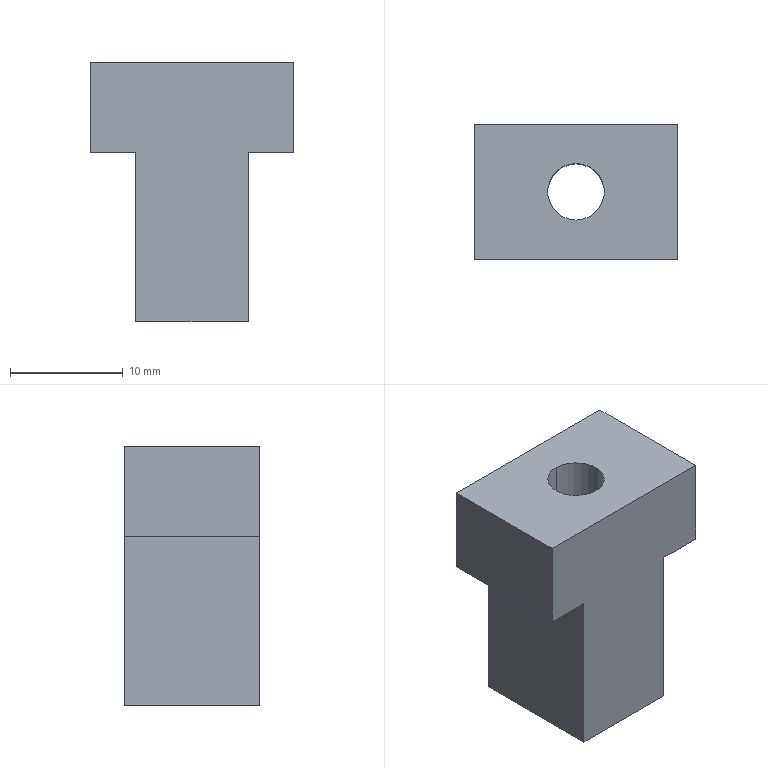Component | SolidWorks | SecondGenerationFour-sidedLabelingFeedingCylinderConnector-1 | 1 solid | 12 faces | box 18 x 12 x 23 mm | volume 3076 mm3 | plane 10 | cylinder 2 | commonest cylinder face diameters 5 x2
build123d program:
from build123d import *

# Parameters (mm, degrees)
SKETCH1_W             = 18
SKETCH1_H             = 8
BOSS_EXTRUDE1_DEPTH   = 6
SKETCH2_W             = 10
SKETCH2_H             = 12
BOSS_EXTRUDE2_DEPTH   = 15
M6_TAPPED_HOLE1_D     = 5
M6_TAPPED_HOLE1_DEPTH = 25
M6_TAPPED_HOLE1_TIP   = 1.502


with BuildPart() as part:
    # Sketch1 → Boss-Extrude1 (new, symmetric)
    with BuildSketch(Plane.XY):
        Rectangle(SKETCH1_W, SKETCH1_H)
    extrude(amount=BOSS_EXTRUDE1_DEPTH, both=True)

    # Sketch2 → Boss-Extrude2 (add)
    with BuildSketch(Plane(origin=(0, 4, 0), x_dir=(1, 0, 0), z_dir=(0, 1, 0))):
        Rectangle(SKETCH2_W, SKETCH2_H)
    extrude(amount=BOSS_EXTRUDE2_DEPTH)

    # M6 Tapped Hole1
    with Locations(Plane(origin=(0, 19, 0), x_dir=(-1, 0, 0), z_dir=(0, 1, 0))):
        with Locations((0, 0)):
            Hole(M6_TAPPED_HOLE1_D / 2, depth=M6_TAPPED_HOLE1_DEPTH)
            with Locations((0, 0, -(M6_TAPPED_HOLE1_DEPTH + M6_TAPPED_HOLE1_TIP / 2))):  # 118° drill point
                Cone(0, M6_TAPPED_HOLE1_D / 2, M6_TAPPED_HOLE1_TIP, mode=Mode.SUBTRACT)


solid = part.part

# Placed as in the assembly
solid = solid.moved(Location((59.973, -16.137, -142.5), (-90, 0, 0)))
STEP:
#1=CARTESIAN_POINT('',(2.361,-0.7337,-5.453));
#2=VERTEX_POINT('',#1);
#3=CARTESIAN_POINT('',(2.361,-0.5369,-5.453));
#4=VERTEX_POINT('',#3);
#5=CARTESIAN_POINT('',(2.361,-0.6353,-5.453));
#6=DIRECTION('',(-0.,-0.,-1.));
#7=DIRECTION('',(0.,1.,0.));
#8=AXIS2_PLACEMENT_3D('',#5,#6,#7);
#9=CIRCLE('',#8,0.09843);
#10=EDGE_CURVE('',#2,#4,#9,.T.);
#11=ORIENTED_EDGE('',*,*,#10,.F.);
#12=CARTESIAN_POINT('',(2.361,-0.7337,-6.358));
#13=VERTEX_POINT('',#12);
#14=CARTESIAN_POINT('',(2.361,-0.7337,-6.358));
#15=DIRECTION('',(-0.,-0.,-1.));
#16=VECTOR('',#15,39.37);
#17=LINE('',#14,#16);
#18=EDGE_CURVE('',#2,#13,#17,.T.);
#19=ORIENTED_EDGE('',*,*,#18,.T.);
#20=CARTESIAN_POINT('',(2.361,-0.5369,-6.358));
#21=VERTEX_POINT('',#20);
#22=CARTESIAN_POINT('',(2.361,-0.6353,-6.358));
#23=DIRECTION('',(-0.,-0.,-1.));
#24=DIRECTION('',(0.,1.,0.));
#25=AXIS2_PLACEMENT_3D('',#22,#23,#24);
#26=CIRCLE('',#25,0.09843);
#27=EDGE_CURVE('',#13,#21,#26,.T.);
#28=ORIENTED_EDGE('',*,*,#27,.T.);
#29=CARTESIAN_POINT('',(2.361,-0.5369,-6.358));
#30=DIRECTION('',(-0.,-0.,-1.));
#31=VECTOR('',#30,39.37);
#32=LINE('',#29,#31);
#33=EDGE_CURVE('',#4,#21,#32,.T.);
#34=ORIENTED_EDGE('',*,*,#33,.F.);
#35=EDGE_LOOP('',(#11,#19,#28,#34));
#36=FACE_OUTER_BOUND('',#35,.T.);
#37=CARTESIAN_POINT('',(2.361,-0.6353,-6.358));
#38=DIRECTION('',(-0.,-0.,-1.));
#39=DIRECTION('',(0.,1.,0.));
#40=AXIS2_PLACEMENT_3D('',#37,#38,#39);
#41=CYLINDRICAL_SURFACE('',#40,0.09843);
#42=ADVANCED_FACE('',(#36),#41,.F.);
#43=CARTESIAN_POINT('',(2.558,-0.3991,-5.768));
#44=VERTEX_POINT('',#43);
#45=CARTESIAN_POINT('',(2.558,-0.8715,-5.768));
#46=VERTEX_POINT('',#45);
#47=CARTESIAN_POINT('',(2.558,-0.3991,-5.768));
#48=DIRECTION('',(-0.,-1.,0.));
#49=VECTOR('',#48,39.37);
#50=LINE('',#47,#49);
#51=EDGE_CURVE('',#44,#46,#50,.T.);
#52=ORIENTED_EDGE('',*,*,#51,.F.);
#53=CARTESIAN_POINT('',(2.715,-0.3991,-5.768));
#54=VERTEX_POINT('',#53);
#55=CARTESIAN_POINT('',(2.007,-0.3991,-5.768));
#56=DIRECTION('',(-1.,0.,0.));
#57=VECTOR('',#56,39.37);
#58=LINE('',#55,#57);
#59=EDGE_CURVE('',#54,#44,#58,.T.);
#60=ORIENTED_EDGE('',*,*,#59,.F.);
#61=CARTESIAN_POINT('',(2.715,-0.8715,-5.768));
#62=VERTEX_POINT('',#61);
#63=CARTESIAN_POINT('',(2.715,-0.3991,-5.768));
#64=DIRECTION('',(-0.,-1.,0.));
#65=VECTOR('',#64,39.37);
#66=LINE('',#63,#65);
#67=EDGE_CURVE('',#54,#62,#66,.T.);
#68=ORIENTED_EDGE('',*,*,#67,.T.);
#69=CARTESIAN_POINT('',(2.007,-0.8715,-5.768));
#70=DIRECTION('',(-1.,0.,0.));
#71=VECTOR('',#70,39.37);
#72=LINE('',#69,#71);
#73=EDGE_CURVE('',#62,#46,#72,.T.);
#74=ORIENTED_EDGE('',*,*,#73,.T.);
#75=EDGE_LOOP('',(#52,#60,#68,#74));
#76=FACE_OUTER_BOUND('',#75,.T.);
#77=CARTESIAN_POINT('',(2.007,-0.3991,-5.768));
#78=DIRECTION('',(0.,0.,1.));
#79=DIRECTION('',(-0.,-1.,0.));
#80=AXIS2_PLACEMENT_3D('',#77,#78,#79);
#81=PLANE('',#80);
#82=ADVANCED_FACE('',(#76),#81,.F.);
#83=CARTESIAN_POINT('',(2.164,-0.8715,-5.768));
#84=VERTEX_POINT('',#83);
#85=CARTESIAN_POINT('',(2.164,-0.3991,-5.768));
#86=VERTEX_POINT('',#85);
#87=CARTESIAN_POINT('',(2.164,-0.3991,-5.768));
#88=DIRECTION('',(0.,1.,-0.));
#89=VECTOR('',#88,39.37);
#90=LINE('',#87,#89);
#91=EDGE_CURVE('',#84,#86,#90,.T.);
#92=ORIENTED_EDGE('',*,*,#91,.F.);
#93=CARTESIAN_POINT('',(2.007,-0.8715,-5.768));
#94=VERTEX_POINT('',#93);
#95=CARTESIAN_POINT('',(2.007,-0.8715,-5.768));
#96=DIRECTION('',(-1.,0.,0.));
#97=VECTOR('',#96,39.37);
#98=LINE('',#95,#97);
#99=EDGE_CURVE('',#84,#94,#98,.T.);
#100=ORIENTED_EDGE('',*,*,#99,.T.);
#101=CARTESIAN_POINT('',(2.007,-0.3991,-5.768));
#102=VERTEX_POINT('',#101);
#103=CARTESIAN_POINT('',(2.007,-0.3991,-5.768));
#104=DIRECTION('',(-0.,-1.,0.));
#105=VECTOR('',#104,39.37);
#106=LINE('',#103,#105);
#107=EDGE_CURVE('',#102,#94,#106,.T.);
#108=ORIENTED_EDGE('',*,*,#107,.F.);
#109=CARTESIAN_POINT('',(2.007,-0.3991,-5.768));
#110=DIRECTION('',(-1.,0.,0.));
#111=VECTOR('',#110,39.37);
#112=LINE('',#109,#111);
#113=EDGE_CURVE('',#86,#102,#112,.T.);
#114=ORIENTED_EDGE('',*,*,#113,.F.);
#115=EDGE_LOOP('',(#92,#100,#108,#114));
#116=FACE_OUTER_BOUND('',#115,.T.);
#117=CARTESIAN_POINT('',(2.007,-0.3991,-5.768));
#118=DIRECTION('',(0.,0.,1.));
#119=DIRECTION('',(-0.,-1.,0.));
#120=AXIS2_PLACEMENT_3D('',#117,#118,#119);
#121=PLANE('',#120);
#122=ADVANCED_FACE('',(#116),#121,.F.);
#123=CARTESIAN_POINT('',(2.715,-0.8715,-5.453));
#124=VERTEX_POINT('',#123);
#125=CARTESIAN_POINT('',(2.715,-0.8715,-5.453));
#126=DIRECTION('',(-0.,-0.,-1.));
#127=VECTOR('',#126,39.37);
#128=LINE('',#125,#127);
#129=EDGE_CURVE('',#124,#62,#128,.T.);
#130=ORIENTED_EDGE('',*,*,#129,.T.);
#131=ORIENTED_EDGE('',*,*,#67,.F.);
#132=CARTESIAN_POINT('',(2.715,-0.3991,-5.453));
#133=VERTEX_POINT('',#132);
#134=CARTESIAN_POINT('',(2.715,-0.3991,-5.453));
#135=DIRECTION('',(-0.,-0.,-1.));
#136=VECTOR('',#135,39.37);
#137=LINE('',#134,#136);
#138=EDGE_CURVE('',#133,#54,#137,.T.);
#139=ORIENTED_EDGE('',*,*,#138,.F.);
#140=CARTESIAN_POINT('',(2.715,-0.3991,-5.453));
#141=DIRECTION('',(-0.,-1.,0.));
#142=VECTOR('',#141,39.37);
#143=LINE('',#140,#142);
#144=EDGE_CURVE('',#133,#124,#143,.T.);
#145=ORIENTED_EDGE('',*,*,#144,.T.);
#146=EDGE_LOOP('',(#130,#131,#139,#145));
#147=FACE_OUTER_BOUND('',#146,.T.);
#148=CARTESIAN_POINT('',(2.715,-0.3991,-5.453));
#149=DIRECTION('',(-1.,0.,0.));
#150=DIRECTION('',(0.,1.,-0.));
#151=AXIS2_PLACEMENT_3D('',#148,#149,#150);
#152=PLANE('',#151);
#153=ADVANCED_FACE('',(#147),#152,.F.);
#154=CARTESIAN_POINT('',(2.007,-0.8715,-5.453));
#155=VERTEX_POINT('',#154);
#156=CARTESIAN_POINT('',(2.007,-0.8715,-5.453));
#157=DIRECTION('',(0.,0.,1.));
#158=VECTOR('',#157,39.37);
#159=LINE('',#156,#158);
#160=EDGE_CURVE('',#94,#155,#159,.T.);
#161=ORIENTED_EDGE('',*,*,#160,.T.);
#162=CARTESIAN_POINT('',(2.007,-0.3991,-5.453));
#163=VERTEX_POINT('',#162);
#164=CARTESIAN_POINT('',(2.007,-0.3991,-5.453));
#165=DIRECTION('',(-0.,-1.,0.));
#166=VECTOR('',#165,39.37);
#167=LINE('',#164,#166);
#168=EDGE_CURVE('',#163,#155,#167,.T.);
#169=ORIENTED_EDGE('',*,*,#168,.F.);
#170=CARTESIAN_POINT('',(2.007,-0.3991,-5.453));
#171=DIRECTION('',(0.,0.,1.));
#172=VECTOR('',#171,39.37);
#173=LINE('',#170,#172);
#174=EDGE_CURVE('',#102,#163,#173,.T.);
#175=ORIENTED_EDGE('',*,*,#174,.F.);
#176=ORIENTED_EDGE('',*,*,#107,.T.);
#177=EDGE_LOOP('',(#161,#169,#175,#176));
#178=FACE_OUTER_BOUND('',#177,.T.);
#179=CARTESIAN_POINT('',(2.007,-0.3991,-5.453));
#180=DIRECTION('',(1.,-0.,-0.));
#181=DIRECTION('',(-0.,-1.,0.));
#182=AXIS2_PLACEMENT_3D('',#179,#180,#181);
#183=PLANE('',#182);
#184=ADVANCED_FACE('',(#178),#183,.F.);
#185=CARTESIAN_POINT('',(2.361,-0.6353,-5.453));
#186=DIRECTION('',(-0.,-0.,-1.));
#187=DIRECTION('',(0.,1.,0.));
#188=AXIS2_PLACEMENT_3D('',#185,#186,#187);
#189=CIRCLE('',#188,0.09843);
#190=EDGE_CURVE('',#4,#2,#189,.T.);
#191=ORIENTED_EDGE('',*,*,#190,.T.);
#192=ORIENTED_EDGE('',*,*,#10,.T.);
#193=EDGE_LOOP('',(#191,#192));
#194=FACE_BOUND('',#193,.T.);
#195=CARTESIAN_POINT('',(2.007,-0.8715,-5.453));
#196=DIRECTION('',(1.,-0.,-0.));
#197=VECTOR('',#196,39.37);
#198=LINE('',#195,#197);
#199=EDGE_CURVE('',#155,#124,#198,.T.);
#200=ORIENTED_EDGE('',*,*,#199,.T.);
#201=ORIENTED_EDGE('',*,*,#144,.F.);
#202=CARTESIAN_POINT('',(2.007,-0.3991,-5.453));
#203=DIRECTION('',(1.,-0.,-0.));
#204=VECTOR('',#203,39.37);
#205=LINE('',#202,#204);
#206=EDGE_CURVE('',#163,#133,#205,.T.);
#207=ORIENTED_EDGE('',*,*,#206,.F.);
#208=ORIENTED_EDGE('',*,*,#168,.T.);
#209=EDGE_LOOP('',(#200,#201,#207,#208));
#210=FACE_OUTER_BOUND('',#209,.T.);
#211=CARTESIAN_POINT('',(2.007,-0.3991,-5.453));
#212=DIRECTION('',(-0.,-0.,-1.));
#213=DIRECTION('',(0.,1.,-0.));
#214=AXIS2_PLACEMENT_3D('',#211,#212,#213);
#215=PLANE('',#214);
#216=ADVANCED_FACE('',(#194,#210),#215,.F.);
#217=ORIENTED_EDGE('',*,*,#138,.T.);
#218=ORIENTED_EDGE('',*,*,#59,.T.);
#219=CARTESIAN_POINT('',(2.558,-0.3991,-6.358));
#220=VERTEX_POINT('',#219);
#221=CARTESIAN_POINT('',(2.558,-0.3991,-6.358));
#222=DIRECTION('',(0.,0.,1.));
#223=VECTOR('',#222,39.37);
#224=LINE('',#221,#223);
#225=EDGE_CURVE('',#220,#44,#224,.T.);
#226=ORIENTED_EDGE('',*,*,#225,.F.);
#227=CARTESIAN_POINT('',(2.164,-0.3991,-6.358));
#228=VERTEX_POINT('',#227);
#229=CARTESIAN_POINT('',(2.164,-0.3991,-6.358));
#230=DIRECTION('',(1.,-0.,-0.));
#231=VECTOR('',#230,39.37);
#232=LINE('',#229,#231);
#233=EDGE_CURVE('',#228,#220,#232,.T.);
#234=ORIENTED_EDGE('',*,*,#233,.F.);
#235=CARTESIAN_POINT('',(2.164,-0.3991,-6.358));
#236=DIRECTION('',(0.,0.,1.));
#237=VECTOR('',#236,39.37);
#238=LINE('',#235,#237);
#239=EDGE_CURVE('',#228,#86,#238,.T.);
#240=ORIENTED_EDGE('',*,*,#239,.T.);
#241=ORIENTED_EDGE('',*,*,#113,.T.);
#242=ORIENTED_EDGE('',*,*,#174,.T.);
#243=ORIENTED_EDGE('',*,*,#206,.T.);
#244=EDGE_LOOP('',(#217,#218,#226,#234,#240,#241,#242,#243));
#245=FACE_OUTER_BOUND('',#244,.T.);
#246=CARTESIAN_POINT('',(2.715,-0.3991,-5.768));
#247=DIRECTION('',(-0.,-1.,0.));
#248=DIRECTION('',(-1.,0.,0.));
#249=AXIS2_PLACEMENT_3D('',#246,#247,#248);
#250=PLANE('',#249);
#251=ADVANCED_FACE('',(#245),#250,.F.);
#252=ORIENTED_EDGE('',*,*,#129,.F.);
#253=ORIENTED_EDGE('',*,*,#199,.F.);
#254=ORIENTED_EDGE('',*,*,#160,.F.);
#255=ORIENTED_EDGE('',*,*,#99,.F.);
#256=CARTESIAN_POINT('',(2.164,-0.8715,-6.358));
#257=VERTEX_POINT('',#256);
#258=CARTESIAN_POINT('',(2.164,-0.8715,-6.358));
#259=DIRECTION('',(0.,0.,1.));
#260=VECTOR('',#259,39.37);
#261=LINE('',#258,#260);
#262=EDGE_CURVE('',#257,#84,#261,.T.);
#263=ORIENTED_EDGE('',*,*,#262,.F.);
#264=CARTESIAN_POINT('',(2.558,-0.8715,-6.358));
#265=VERTEX_POINT('',#264);
#266=CARTESIAN_POINT('',(2.164,-0.8715,-6.358));
#267=DIRECTION('',(-1.,0.,0.));
#268=VECTOR('',#267,39.37);
#269=LINE('',#266,#268);
#270=EDGE_CURVE('',#265,#257,#269,.T.);
#271=ORIENTED_EDGE('',*,*,#270,.F.);
#272=CARTESIAN_POINT('',(2.558,-0.8715,-6.358));
#273=DIRECTION('',(0.,0.,1.));
#274=VECTOR('',#273,39.37);
#275=LINE('',#272,#274);
#276=EDGE_CURVE('',#265,#46,#275,.T.);
#277=ORIENTED_EDGE('',*,*,#276,.T.);
#278=ORIENTED_EDGE('',*,*,#73,.F.);
#279=EDGE_LOOP('',(#252,#253,#254,#255,#263,#271,#277,#278));
#280=FACE_OUTER_BOUND('',#279,.T.);
#281=CARTESIAN_POINT('',(2.715,-0.8715,-5.768));
#282=DIRECTION('',(-0.,-1.,0.));
#283=DIRECTION('',(-1.,0.,0.));
#284=AXIS2_PLACEMENT_3D('',#281,#282,#283);
#285=PLANE('',#284);
#286=ADVANCED_FACE('',(#280),#285,.T.);
#287=ORIENTED_EDGE('',*,*,#51,.T.);
#288=ORIENTED_EDGE('',*,*,#276,.F.);
#289=CARTESIAN_POINT('',(2.558,-0.3991,-6.358));
#290=DIRECTION('',(-0.,-1.,0.));
#291=VECTOR('',#290,39.37);
#292=LINE('',#289,#291);
#293=EDGE_CURVE('',#220,#265,#292,.T.);
#294=ORIENTED_EDGE('',*,*,#293,.F.);
#295=ORIENTED_EDGE('',*,*,#225,.T.);
#296=EDGE_LOOP('',(#287,#288,#294,#295));
#297=FACE_OUTER_BOUND('',#296,.T.);
#298=CARTESIAN_POINT('',(2.558,-0.3991,-6.358));
#299=DIRECTION('',(-1.,0.,0.));
#300=DIRECTION('',(0.,1.,-0.));
#301=AXIS2_PLACEMENT_3D('',#298,#299,#300);
#302=PLANE('',#301);
#303=ADVANCED_FACE('',(#297),#302,.F.);
#304=ORIENTED_EDGE('',*,*,#91,.T.);
#305=ORIENTED_EDGE('',*,*,#239,.F.);
#306=CARTESIAN_POINT('',(2.164,-0.3991,-6.358));
#307=DIRECTION('',(0.,1.,-0.));
#308=VECTOR('',#307,39.37);
#309=LINE('',#306,#308);
#310=EDGE_CURVE('',#257,#228,#309,.T.);
#311=ORIENTED_EDGE('',*,*,#310,.F.);
#312=ORIENTED_EDGE('',*,*,#262,.T.);
#313=EDGE_LOOP('',(#304,#305,#311,#312));
#314=FACE_OUTER_BOUND('',#313,.T.);
#315=CARTESIAN_POINT('',(2.164,-0.3991,-6.358));
#316=DIRECTION('',(1.,-0.,-0.));
#317=DIRECTION('',(-0.,-1.,0.));
#318=AXIS2_PLACEMENT_3D('',#315,#316,#317);
#319=PLANE('',#318);
#320=ADVANCED_FACE('',(#314),#319,.F.);
#321=CARTESIAN_POINT('',(2.361,-0.6353,-6.358));
#322=DIRECTION('',(-0.,-0.,-1.));
#323=DIRECTION('',(0.,1.,0.));
#324=AXIS2_PLACEMENT_3D('',#321,#322,#323);
#325=CIRCLE('',#324,0.09843);
#326=EDGE_CURVE('',#21,#13,#325,.T.);
#327=ORIENTED_EDGE('',*,*,#326,.F.);
#328=ORIENTED_EDGE('',*,*,#27,.F.);
#329=EDGE_LOOP('',(#327,#328));
#330=FACE_BOUND('',#329,.T.);
#331=ORIENTED_EDGE('',*,*,#293,.T.);
#332=ORIENTED_EDGE('',*,*,#270,.T.);
#333=ORIENTED_EDGE('',*,*,#310,.T.);
#334=ORIENTED_EDGE('',*,*,#233,.T.);
#335=EDGE_LOOP('',(#331,#332,#333,#334));
#336=FACE_OUTER_BOUND('',#335,.T.);
#337=CARTESIAN_POINT('',(2.558,-0.8715,-6.358));
#338=DIRECTION('',(0.,0.,1.));
#339=DIRECTION('',(-0.,-1.,0.));
#340=AXIS2_PLACEMENT_3D('',#337,#338,#339);
#341=PLANE('',#340);
#342=ADVANCED_FACE('',(#330,#336),#341,.F.);
#343=ORIENTED_EDGE('',*,*,#18,.F.);
#344=ORIENTED_EDGE('',*,*,#190,.F.);
#345=ORIENTED_EDGE('',*,*,#33,.T.);
#346=ORIENTED_EDGE('',*,*,#326,.T.);
#347=EDGE_LOOP('',(#343,#344,#345,#346));
#348=FACE_OUTER_BOUND('',#347,.T.);
#349=CARTESIAN_POINT('',(2.361,-0.6353,-6.358));
#350=DIRECTION('',(-0.,-0.,-1.));
#351=DIRECTION('',(0.,1.,0.));
#352=AXIS2_PLACEMENT_3D('',#349,#350,#351);
#353=CYLINDRICAL_SURFACE('',#352,0.09843);
#354=ADVANCED_FACE('',(#348),#353,.F.);
#355=CLOSED_SHELL('',(#42,#82,#122,#153,#184,#216,#251,#286,#303,#320,#342,#354));
#356=MANIFOLD_SOLID_BREP('',#355);
#357=CARTESIAN_POINT('',(0.,0.,0.));
#358=DIRECTION('',(0.,0.,1.));
#359=DIRECTION('',(1.,0.,0.));
#360=AXIS2_PLACEMENT_3D('',#357,#358,#359);
#361=(LENGTH_UNIT()NAMED_UNIT(*)SI_UNIT($,.METRE.));
#362=LENGTH_MEASURE_WITH_UNIT(LENGTH_MEASURE(0.0254),#361);
#363=DIMENSIONAL_EXPONENTS(1.,0.,0.,0.,0.,0.,0.);
#364=(CONVERSION_BASED_UNIT('',#362)LENGTH_UNIT()NAMED_UNIT(#363));
#365=UNCERTAINTY_MEASURE_WITH_UNIT(LENGTH_MEASURE(0.00001),#364,'','');
#366=(NAMED_UNIT(*)PLANE_ANGLE_UNIT()SI_UNIT($,.RADIAN.));
#367=(NAMED_UNIT(*)SI_UNIT($,.STERADIAN.)SOLID_ANGLE_UNIT());
#368=(GEOMETRIC_REPRESENTATION_CONTEXT(3)GLOBAL_UNCERTAINTY_ASSIGNED_CONTEXT((#365))GLOBAL_UNIT_ASSIGNED_CONTEXT((#364,#366,#367))REPRESENTATION_CONTEXT('',''));
#369=ADVANCED_BREP_SHAPE_REPRESENTATION('',(#356,#360),#368);
#370=COLOUR_RGB('',0.7922,0.8196,0.9333);
#371=FILL_AREA_STYLE_COLOUR('',#370);
#372=FILL_AREA_STYLE('',(#371));
#373=SURFACE_STYLE_FILL_AREA(#372);
#374=SURFACE_SIDE_STYLE('',(#373));
#375=SURFACE_STYLE_USAGE(.BOTH.,#374);
#376=PRESENTATION_STYLE_ASSIGNMENT((#375));
#377=STYLED_ITEM('',(#376),#356);
#378=(LENGTH_UNIT()NAMED_UNIT(*)SI_UNIT($,.METRE.));
#379=LENGTH_MEASURE_WITH_UNIT(LENGTH_MEASURE(0.0254),#378);
#380=DIMENSIONAL_EXPONENTS(1.,0.,0.,0.,0.,0.,0.);
#381=(CONVERSION_BASED_UNIT('',#379)LENGTH_UNIT()NAMED_UNIT(#380));
#382=UNCERTAINTY_MEASURE_WITH_UNIT(LENGTH_MEASURE(0.00001),#381,'','');
#383=(NAMED_UNIT(*)PLANE_ANGLE_UNIT()SI_UNIT($,.RADIAN.));
#384=(NAMED_UNIT(*)SI_UNIT($,.STERADIAN.)SOLID_ANGLE_UNIT());
#385=(GEOMETRIC_REPRESENTATION_CONTEXT(3)GLOBAL_UNCERTAINTY_ASSIGNED_CONTEXT((#382))GLOBAL_UNIT_ASSIGNED_CONTEXT((#381,#383,#384))REPRESENTATION_CONTEXT('',''));
#386=MECHANICAL_DESIGN_GEOMETRIC_PRESENTATION_REPRESENTATION('',(#377),#385);
#387=PRESENTATION_LAYER_ASSIGNMENT('','',(#377));